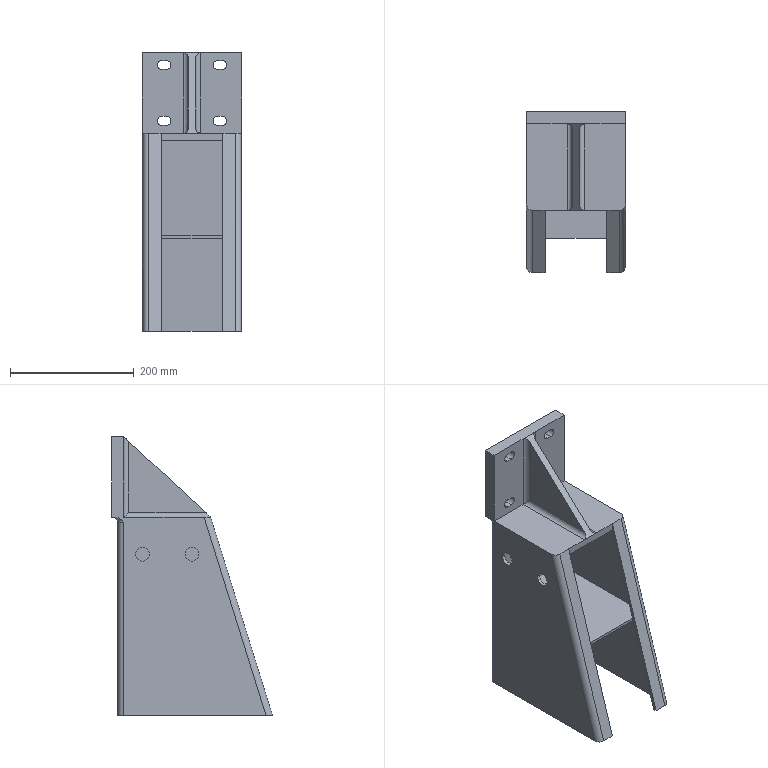Component | SolidWorks | 011FrameLowerElectrodeWeldedPart-1 | 1 solid | 70 faces | volume 1839346 mm3 | plane 39 | cylinder 29 | torus 2 | commonest cylinder face diameters 14 x8 10 x6 16 x5 22 x4 20 x4 60 x2 | material Plain Carbon Steel